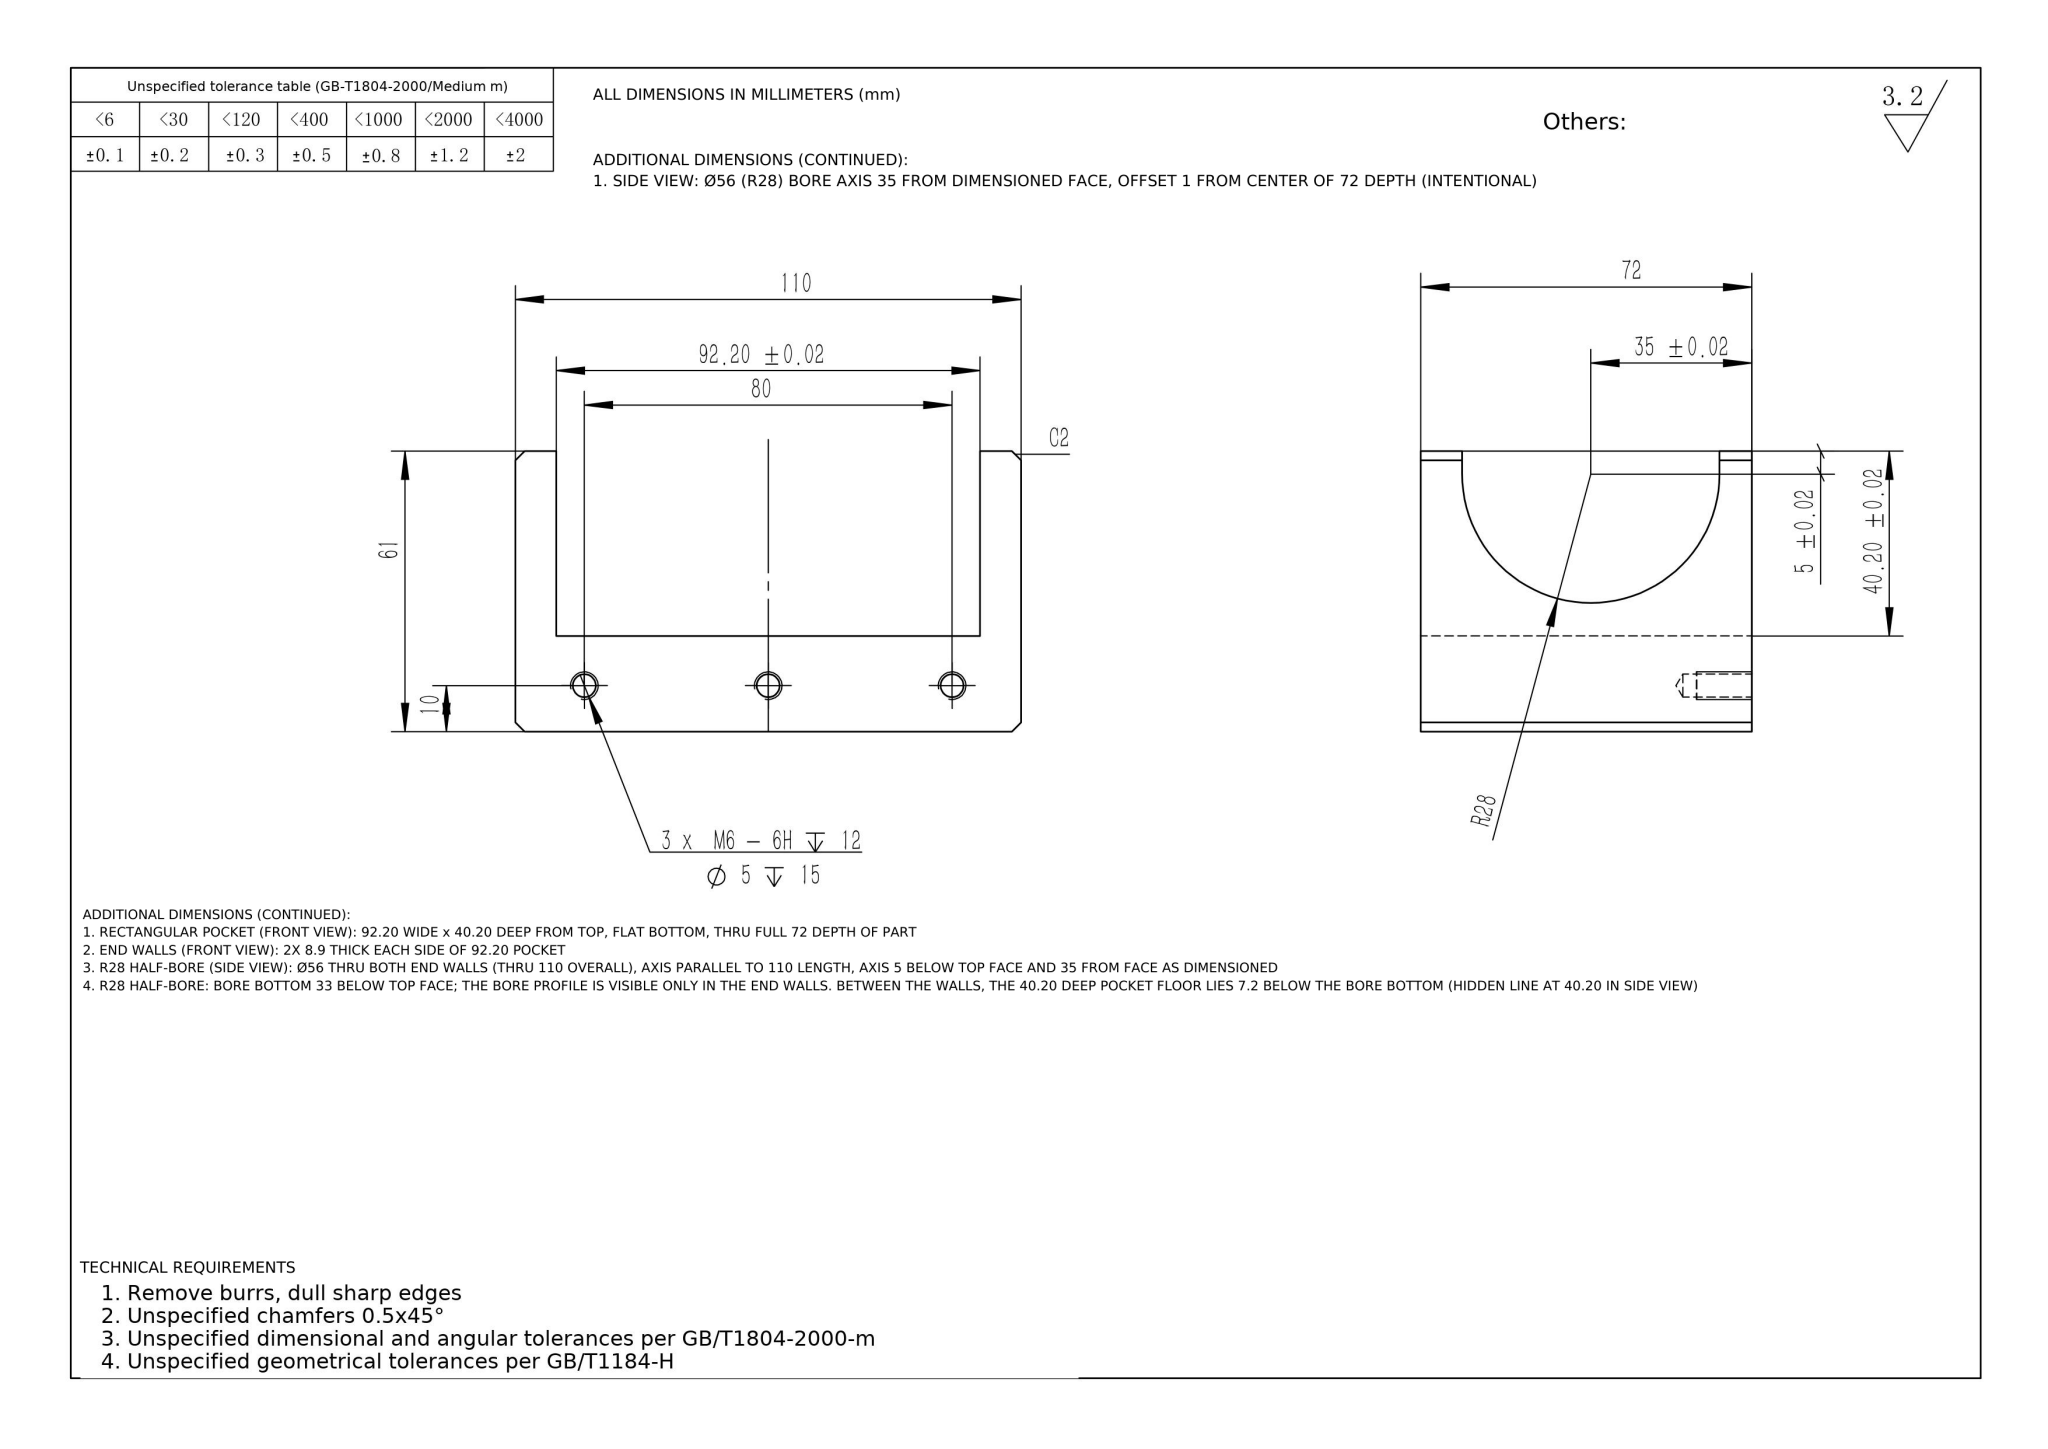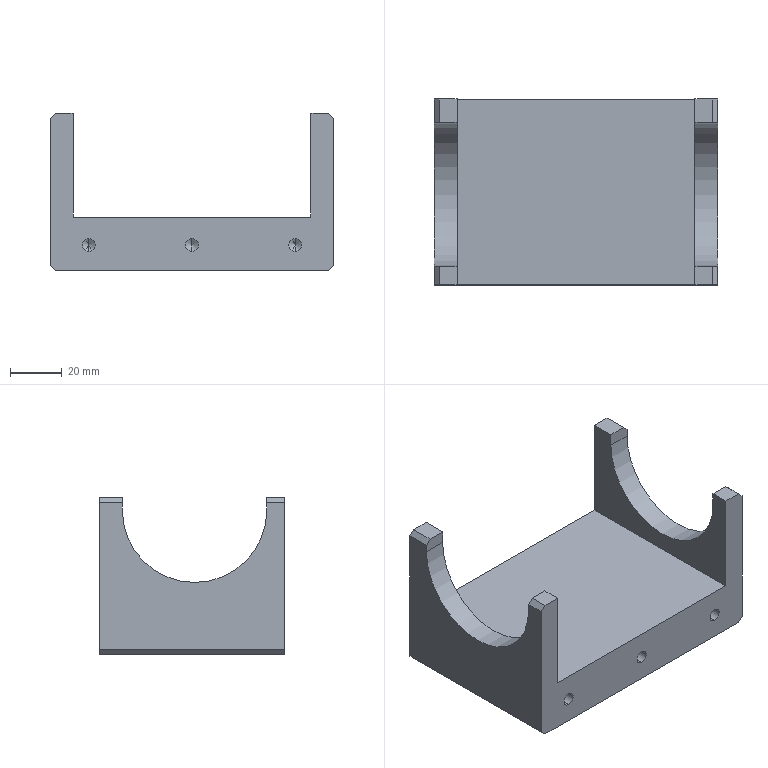Part | NX | mm | 1 solid | 36 faces | box 110 x 72 x 61 mm | volume 188086 mm3 | plane 22 | cylinder 8 | cone 6 | commonest cylinder face diameters 5 x6 56 x2